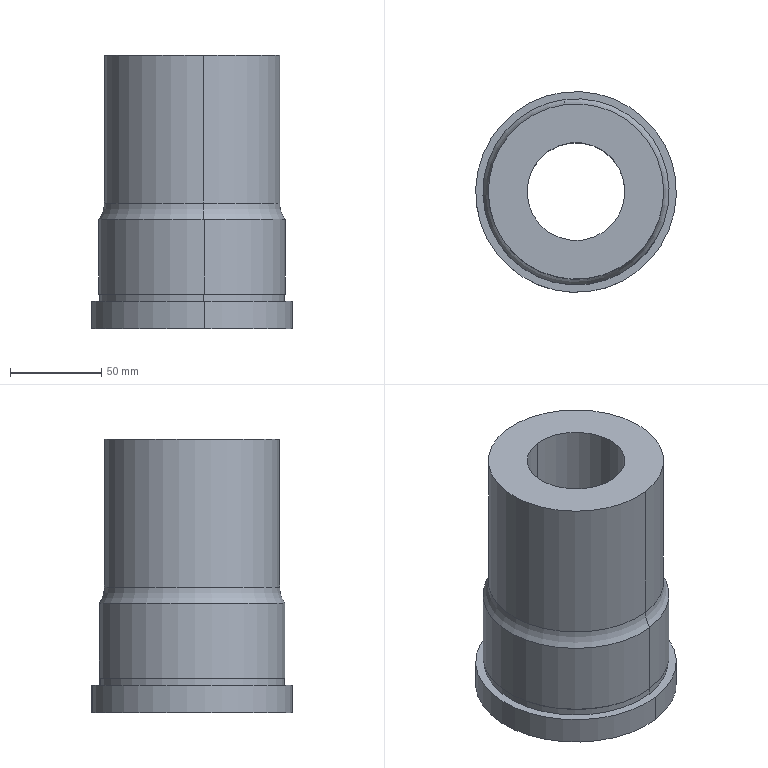Component | SolidWorks | 2-1 | 1 solid | 19 faces | box 110 x 110 x 150 mm | volume 797623 mm3 | cylinder 12 | plane 5 | torus 2 | commonest cylinder face diameters 101 x2 60.5 x2 96.05 x2 102 x2 110 x2 53.65 x2
STEP:
#1=COLOUR_RGB('',0.7922,0.8196,0.9333);
#2=FILL_AREA_STYLE_COLOUR('',#1);
#3=FILL_AREA_STYLE('',(#2));
#4=SURFACE_STYLE_FILL_AREA(#3);
#5=SURFACE_SIDE_STYLE('',(#4));
#6=SURFACE_STYLE_USAGE(.BOTH.,#5);
#7=PRESENTATION_STYLE_ASSIGNMENT((#6));
#8=CARTESIAN_POINT('',(-0.2594,1.991,-7.323));
#9=VERTEX_POINT('',#8);
#10=CARTESIAN_POINT('',(-0.2443,1.875,-6.97));
#11=VERTEX_POINT('',#10);
#12=CARTESIAN_POINT('',(-0.3206,2.461,-6.97));
#13=DIRECTION('',(-0.9916,-0.1292,0.));
#14=DIRECTION('',(-0.1292,0.9916,0.));
#15=AXIS2_PLACEMENT_3D('',#12,#13,#14);
#16=CIRCLE('',#15,0.5906);
#17=EDGE_CURVE('',#9,#11,#16,.T.);
#18=ORIENTED_EDGE('',*,*,#17,.F.);
#19=CARTESIAN_POINT('',(0.2594,-1.991,-7.323));
#20=VERTEX_POINT('',#19);
#21=CARTESIAN_POINT('',(-0.,0.,-7.323));
#22=DIRECTION('',(0.,0.,1.));
#23=DIRECTION('',(-0.1292,0.9916,0.));
#24=AXIS2_PLACEMENT_3D('',#21,#22,#23);
#25=CIRCLE('',#24,2.008);
#26=EDGE_CURVE('',#9,#20,#25,.T.);
#27=ORIENTED_EDGE('',*,*,#26,.T.);
#28=CARTESIAN_POINT('',(0.2443,-1.875,-6.97));
#29=VERTEX_POINT('',#28);
#30=CARTESIAN_POINT('',(0.3206,-2.461,-6.97));
#31=DIRECTION('',(0.9916,0.1292,-0.));
#32=DIRECTION('',(0.1292,-0.9916,0.));
#33=AXIS2_PLACEMENT_3D('',#30,#31,#32);
#34=CIRCLE('',#33,0.5906);
#35=EDGE_CURVE('',#20,#29,#34,.T.);
#36=ORIENTED_EDGE('',*,*,#35,.T.);
#37=CARTESIAN_POINT('',(-0.,0.,-6.97));
#38=DIRECTION('',(0.,0.,1.));
#39=DIRECTION('',(0.1292,-0.9916,0.));
#40=AXIS2_PLACEMENT_3D('',#37,#38,#39);
#41=CIRCLE('',#40,1.891);
#42=EDGE_CURVE('',#11,#29,#41,.T.);
#43=ORIENTED_EDGE('',*,*,#42,.F.);
#44=EDGE_LOOP('',(#18,#27,#36,#43));
#45=FACE_OUTER_BOUND('',#44,.T.);
#46=CARTESIAN_POINT('',(-0.,0.,-6.97));
#47=DIRECTION('',(-0.,-0.,-1.));
#48=DIRECTION('',(0.1292,-0.9916,0.));
#49=AXIS2_PLACEMENT_3D('',#46,#47,#48);
#50=TOROIDAL_SURFACE('',#49,2.481,0.5906);
#51=ADVANCED_FACE('',(#45),#50,.F.);
#52=CARTESIAN_POINT('',(-0.2569,1.972,-8.937));
#53=VERTEX_POINT('',#52);
#54=CARTESIAN_POINT('',(-0.2569,1.972,-9.094));
#55=VERTEX_POINT('',#54);
#56=CARTESIAN_POINT('',(-0.2569,1.972,-8.937));
#57=DIRECTION('',(-0.,-0.,-1.));
#58=VECTOR('',#57,39.37);
#59=LINE('',#56,#58);
#60=EDGE_CURVE('',#53,#55,#59,.T.);
#61=ORIENTED_EDGE('',*,*,#60,.F.);
#62=CARTESIAN_POINT('',(0.2569,-1.972,-8.937));
#63=VERTEX_POINT('',#62);
#64=CARTESIAN_POINT('',(-0.,-0.,-8.937));
#65=DIRECTION('',(0.,0.,1.));
#66=DIRECTION('',(-0.1292,0.9916,0.));
#67=AXIS2_PLACEMENT_3D('',#64,#65,#66);
#68=CIRCLE('',#67,1.988);
#69=EDGE_CURVE('',#63,#53,#68,.T.);
#70=ORIENTED_EDGE('',*,*,#69,.F.);
#71=CARTESIAN_POINT('',(0.2569,-1.972,-9.094));
#72=VERTEX_POINT('',#71);
#73=CARTESIAN_POINT('',(0.2569,-1.972,-8.937));
#74=DIRECTION('',(-0.,-0.,-1.));
#75=VECTOR('',#74,39.37);
#76=LINE('',#73,#75);
#77=EDGE_CURVE('',#63,#72,#76,.T.);
#78=ORIENTED_EDGE('',*,*,#77,.T.);
#79=CARTESIAN_POINT('',(-0.,-0.,-9.094));
#80=DIRECTION('',(0.,0.,1.));
#81=DIRECTION('',(-0.1292,0.9916,0.));
#82=AXIS2_PLACEMENT_3D('',#79,#80,#81);
#83=CIRCLE('',#82,1.988);
#84=EDGE_CURVE('',#72,#55,#83,.T.);
#85=ORIENTED_EDGE('',*,*,#84,.T.);
#86=EDGE_LOOP('',(#61,#70,#78,#85));
#87=FACE_OUTER_BOUND('',#86,.T.);
#88=CARTESIAN_POINT('',(-0.,-0.,-8.937));
#89=DIRECTION('',(-0.,-0.,-1.));
#90=DIRECTION('',(0.1292,-0.9916,0.));
#91=AXIS2_PLACEMENT_3D('',#88,#89,#90);
#92=CYLINDRICAL_SURFACE('',#91,1.988);
#93=ADVANCED_FACE('',(#87),#92,.T.);
#94=ORIENTED_EDGE('',*,*,#69,.T.);
#95=CARTESIAN_POINT('',(-0.,-0.,-8.937));
#96=DIRECTION('',(0.,0.,1.));
#97=DIRECTION('',(-0.1292,0.9916,0.));
#98=AXIS2_PLACEMENT_3D('',#95,#96,#97);
#99=CIRCLE('',#98,1.988);
#100=EDGE_CURVE('',#53,#63,#99,.T.);
#101=ORIENTED_EDGE('',*,*,#100,.T.);
#102=EDGE_LOOP('',(#94,#101));
#103=FACE_BOUND('',#102,.T.);
#104=CARTESIAN_POINT('',(-0.2594,1.991,-8.937));
#105=VERTEX_POINT('',#104);
#106=CARTESIAN_POINT('',(0.2594,-1.991,-8.937));
#107=VERTEX_POINT('',#106);
#108=CARTESIAN_POINT('',(-0.,-0.,-8.937));
#109=DIRECTION('',(0.,0.,1.));
#110=DIRECTION('',(-0.1292,0.9916,0.));
#111=AXIS2_PLACEMENT_3D('',#108,#109,#110);
#112=CIRCLE('',#111,2.008);
#113=EDGE_CURVE('',#105,#107,#112,.T.);
#114=ORIENTED_EDGE('',*,*,#113,.F.);
#115=CARTESIAN_POINT('',(-0.,-0.,-8.937));
#116=DIRECTION('',(0.,0.,1.));
#117=DIRECTION('',(-0.1292,0.9916,0.));
#118=AXIS2_PLACEMENT_3D('',#115,#116,#117);
#119=CIRCLE('',#118,2.008);
#120=EDGE_CURVE('',#107,#105,#119,.T.);
#121=ORIENTED_EDGE('',*,*,#120,.F.);
#122=EDGE_LOOP('',(#114,#121));
#123=FACE_OUTER_BOUND('',#122,.T.);
#124=CARTESIAN_POINT('',(-0.,-0.,-8.937));
#125=DIRECTION('',(0.,0.,1.));
#126=DIRECTION('',(-0.1292,0.9916,-0.));
#127=AXIS2_PLACEMENT_3D('',#124,#125,#126);
#128=PLANE('',#127);
#129=ADVANCED_FACE('',(#103,#123),#128,.F.);
#130=CARTESIAN_POINT('',(-0.1539,1.181,-7.913));
#131=VERTEX_POINT('',#130);
#132=CARTESIAN_POINT('',(-0.1539,1.181,-9.685));
#133=VERTEX_POINT('',#132);
#134=CARTESIAN_POINT('',(-0.1539,1.181,-7.913));
#135=DIRECTION('',(-0.,-0.,-1.));
#136=VECTOR('',#135,39.37);
#137=LINE('',#134,#136);
#138=EDGE_CURVE('',#131,#133,#137,.T.);
#139=ORIENTED_EDGE('',*,*,#138,.F.);
#140=CARTESIAN_POINT('',(0.1539,-1.181,-7.913));
#141=VERTEX_POINT('',#140);
#142=CARTESIAN_POINT('',(-0.,-0.,-7.913));
#143=DIRECTION('',(-0.,-0.,-1.));
#144=DIRECTION('',(0.1292,-0.9916,0.));
#145=AXIS2_PLACEMENT_3D('',#142,#143,#144);
#146=CIRCLE('',#145,1.191);
#147=EDGE_CURVE('',#141,#131,#146,.T.);
#148=ORIENTED_EDGE('',*,*,#147,.F.);
#149=CARTESIAN_POINT('',(0.1539,-1.181,-9.685));
#150=VERTEX_POINT('',#149);
#151=CARTESIAN_POINT('',(0.1539,-1.181,-7.913));
#152=DIRECTION('',(-0.,-0.,-1.));
#153=VECTOR('',#152,39.37);
#154=LINE('',#151,#153);
#155=EDGE_CURVE('',#141,#150,#154,.T.);
#156=ORIENTED_EDGE('',*,*,#155,.T.);
#157=CARTESIAN_POINT('',(-0.,-0.,-9.685));
#158=DIRECTION('',(-0.,-0.,-1.));
#159=DIRECTION('',(0.1292,-0.9916,0.));
#160=AXIS2_PLACEMENT_3D('',#157,#158,#159);
#161=CIRCLE('',#160,1.191);
#162=EDGE_CURVE('',#150,#133,#161,.T.);
#163=ORIENTED_EDGE('',*,*,#162,.T.);
#164=EDGE_LOOP('',(#139,#148,#156,#163));
#165=FACE_OUTER_BOUND('',#164,.T.);
#166=CARTESIAN_POINT('',(-0.,-0.,-7.913));
#167=DIRECTION('',(-0.,-0.,-1.));
#168=DIRECTION('',(0.1292,-0.9916,0.));
#169=AXIS2_PLACEMENT_3D('',#166,#167,#168);
#170=CYLINDRICAL_SURFACE('',#169,1.191);
#171=ADVANCED_FACE('',(#165),#170,.F.);
#172=CARTESIAN_POINT('',(-0.1364,1.047,-7.913));
#173=VERTEX_POINT('',#172);
#174=CARTESIAN_POINT('',(0.1364,-1.047,-7.913));
#175=VERTEX_POINT('',#174);
#176=CARTESIAN_POINT('',(-0.,-0.,-7.913));
#177=DIRECTION('',(0.,0.,1.));
#178=DIRECTION('',(0.1292,-0.9916,0.));
#179=AXIS2_PLACEMENT_3D('',#176,#177,#178);
#180=CIRCLE('',#179,1.056);
#181=EDGE_CURVE('',#173,#175,#180,.T.);
#182=ORIENTED_EDGE('',*,*,#181,.T.);
#183=CARTESIAN_POINT('',(-0.,-0.,-7.913));
#184=DIRECTION('',(0.,0.,1.));
#185=DIRECTION('',(0.1292,-0.9916,0.));
#186=AXIS2_PLACEMENT_3D('',#183,#184,#185);
#187=CIRCLE('',#186,1.056);
#188=EDGE_CURVE('',#175,#173,#187,.T.);
#189=ORIENTED_EDGE('',*,*,#188,.T.);
#190=EDGE_LOOP('',(#182,#189));
#191=FACE_BOUND('',#190,.T.);
#192=ORIENTED_EDGE('',*,*,#147,.T.);
#193=CARTESIAN_POINT('',(-0.,-0.,-7.913));
#194=DIRECTION('',(-0.,-0.,-1.));
#195=DIRECTION('',(0.1292,-0.9916,0.));
#196=AXIS2_PLACEMENT_3D('',#193,#194,#195);
#197=CIRCLE('',#196,1.191);
#198=EDGE_CURVE('',#131,#141,#197,.T.);
#199=ORIENTED_EDGE('',*,*,#198,.T.);
#200=EDGE_LOOP('',(#192,#199));
#201=FACE_OUTER_BOUND('',#200,.T.);
#202=CARTESIAN_POINT('',(-0.,-0.,-7.913));
#203=DIRECTION('',(-0.,-0.,-1.));
#204=DIRECTION('',(-0.9916,-0.1292,0.));
#205=AXIS2_PLACEMENT_3D('',#202,#203,#204);
#206=PLANE('',#205);
#207=ADVANCED_FACE('',(#191,#201),#206,.T.);
#208=CARTESIAN_POINT('',(0.2443,-1.875,-3.78));
#209=VERTEX_POINT('',#208);
#210=CARTESIAN_POINT('',(0.2443,-1.875,-3.78));
#211=DIRECTION('',(0.,0.,1.));
#212=VECTOR('',#211,39.37);
#213=LINE('',#210,#212);
#214=EDGE_CURVE('',#29,#209,#213,.T.);
#215=ORIENTED_EDGE('',*,*,#214,.F.);
#216=CARTESIAN_POINT('',(-0.,0.,-6.97));
#217=DIRECTION('',(0.,0.,1.));
#218=DIRECTION('',(0.1292,-0.9916,0.));
#219=AXIS2_PLACEMENT_3D('',#216,#217,#218);
#220=CIRCLE('',#219,1.891);
#221=EDGE_CURVE('',#29,#11,#220,.T.);
#222=ORIENTED_EDGE('',*,*,#221,.T.);
#223=CARTESIAN_POINT('',(-0.2443,1.875,-3.78));
#224=VERTEX_POINT('',#223);
#225=CARTESIAN_POINT('',(-0.2443,1.875,-3.78));
#226=DIRECTION('',(0.,0.,1.));
#227=VECTOR('',#226,39.37);
#228=LINE('',#225,#227);
#229=EDGE_CURVE('',#11,#224,#228,.T.);
#230=ORIENTED_EDGE('',*,*,#229,.T.);
#231=CARTESIAN_POINT('',(-0.,0.,-3.78));
#232=DIRECTION('',(0.,0.,1.));
#233=DIRECTION('',(-0.1292,0.9916,0.));
#234=AXIS2_PLACEMENT_3D('',#231,#232,#233);
#235=CIRCLE('',#234,1.891);
#236=EDGE_CURVE('',#209,#224,#235,.T.);
#237=ORIENTED_EDGE('',*,*,#236,.F.);
#238=EDGE_LOOP('',(#215,#222,#230,#237));
#239=FACE_OUTER_BOUND('',#238,.T.);
#240=CARTESIAN_POINT('',(-0.,0.,-3.78));
#241=DIRECTION('',(0.,0.,1.));
#242=DIRECTION('',(-0.1292,0.9916,0.));
#243=AXIS2_PLACEMENT_3D('',#240,#241,#242);
#244=CYLINDRICAL_SURFACE('',#243,1.891);
#245=ADVANCED_FACE('',(#239),#244,.T.);
#246=CARTESIAN_POINT('',(0.2594,-1.991,-3.78));
#247=DIRECTION('',(0.,0.,1.));
#248=VECTOR('',#247,39.37);
#249=LINE('',#246,#248);
#250=EDGE_CURVE('',#107,#20,#249,.T.);
#251=ORIENTED_EDGE('',*,*,#250,.F.);
#252=ORIENTED_EDGE('',*,*,#120,.T.);
#253=CARTESIAN_POINT('',(-0.2594,1.991,-3.78));
#254=DIRECTION('',(0.,0.,1.));
#255=VECTOR('',#254,39.37);
#256=LINE('',#253,#255);
#257=EDGE_CURVE('',#105,#9,#256,.T.);
#258=ORIENTED_EDGE('',*,*,#257,.T.);
#259=CARTESIAN_POINT('',(-0.,0.,-7.323));
#260=DIRECTION('',(0.,0.,1.));
#261=DIRECTION('',(-0.1292,0.9916,0.));
#262=AXIS2_PLACEMENT_3D('',#259,#260,#261);
#263=CIRCLE('',#262,2.008);
#264=EDGE_CURVE('',#20,#9,#263,.T.);
#265=ORIENTED_EDGE('',*,*,#264,.F.);
#266=EDGE_LOOP('',(#251,#252,#258,#265));
#267=FACE_OUTER_BOUND('',#266,.T.);
#268=CARTESIAN_POINT('',(-0.,0.,-3.78));
#269=DIRECTION('',(0.,0.,1.));
#270=DIRECTION('',(-0.1292,0.9916,0.));
#271=AXIS2_PLACEMENT_3D('',#268,#269,#270);
#272=CYLINDRICAL_SURFACE('',#271,2.008);
#273=ADVANCED_FACE('',(#267),#272,.T.);
#274=ORIENTED_EDGE('',*,*,#84,.F.);
#275=CARTESIAN_POINT('',(-0.,-0.,-9.094));
#276=DIRECTION('',(0.,0.,1.));
#277=DIRECTION('',(-0.1292,0.9916,0.));
#278=AXIS2_PLACEMENT_3D('',#275,#276,#277);
#279=CIRCLE('',#278,1.988);
#280=EDGE_CURVE('',#55,#72,#279,.T.);
#281=ORIENTED_EDGE('',*,*,#280,.F.);
#282=EDGE_LOOP('',(#274,#281));
#283=FACE_BOUND('',#282,.T.);
#284=CARTESIAN_POINT('',(-0.2797,2.147,-9.094));
#285=VERTEX_POINT('',#284);
#286=CARTESIAN_POINT('',(0.2797,-2.147,-9.094));
#287=VERTEX_POINT('',#286);
#288=CARTESIAN_POINT('',(-0.,-0.,-9.094));
#289=DIRECTION('',(0.,0.,1.));
#290=DIRECTION('',(-0.1292,0.9916,0.));
#291=AXIS2_PLACEMENT_3D('',#288,#289,#290);
#292=CIRCLE('',#291,2.165);
#293=EDGE_CURVE('',#285,#287,#292,.T.);
#294=ORIENTED_EDGE('',*,*,#293,.T.);
#295=CARTESIAN_POINT('',(-0.,-0.,-9.094));
#296=DIRECTION('',(0.,0.,1.));
#297=DIRECTION('',(-0.1292,0.9916,0.));
#298=AXIS2_PLACEMENT_3D('',#295,#296,#297);
#299=CIRCLE('',#298,2.165);
#300=EDGE_CURVE('',#287,#285,#299,.T.);
#301=ORIENTED_EDGE('',*,*,#300,.T.);
#302=EDGE_LOOP('',(#294,#301));
#303=FACE_OUTER_BOUND('',#302,.T.);
#304=CARTESIAN_POINT('',(-2.147,-0.2797,-9.094));
#305=DIRECTION('',(0.,0.,1.));
#306=DIRECTION('',(-0.1292,0.9916,-0.));
#307=AXIS2_PLACEMENT_3D('',#304,#305,#306);
#308=PLANE('',#307);
#309=ADVANCED_FACE('',(#283,#303),#308,.T.);
#310=CARTESIAN_POINT('',(0.2797,-2.147,-9.685));
#311=VERTEX_POINT('',#310);
#312=CARTESIAN_POINT('',(0.2797,-2.147,-3.78));
#313=DIRECTION('',(0.,0.,1.));
#314=VECTOR('',#313,39.37);
#315=LINE('',#312,#314);
#316=EDGE_CURVE('',#311,#287,#315,.T.);
#317=ORIENTED_EDGE('',*,*,#316,.F.);
#318=CARTESIAN_POINT('',(-0.2797,2.147,-9.685));
#319=VERTEX_POINT('',#318);
#320=CARTESIAN_POINT('',(-0.,-0.,-9.685));
#321=DIRECTION('',(0.,0.,1.));
#322=DIRECTION('',(-0.1292,0.9916,0.));
#323=AXIS2_PLACEMENT_3D('',#320,#321,#322);
#324=CIRCLE('',#323,2.165);
#325=EDGE_CURVE('',#311,#319,#324,.T.);
#326=ORIENTED_EDGE('',*,*,#325,.T.);
#327=CARTESIAN_POINT('',(-0.2797,2.147,-3.78));
#328=DIRECTION('',(0.,0.,1.));
#329=VECTOR('',#328,39.37);
#330=LINE('',#327,#329);
#331=EDGE_CURVE('',#319,#285,#330,.T.);
#332=ORIENTED_EDGE('',*,*,#331,.T.);
#333=ORIENTED_EDGE('',*,*,#300,.F.);
#334=EDGE_LOOP('',(#317,#326,#332,#333));
#335=FACE_OUTER_BOUND('',#334,.T.);
#336=CARTESIAN_POINT('',(-0.,0.,-3.78));
#337=DIRECTION('',(0.,0.,1.));
#338=DIRECTION('',(-0.1292,0.9916,0.));
#339=AXIS2_PLACEMENT_3D('',#336,#337,#338);
#340=CYLINDRICAL_SURFACE('',#339,2.165);
#341=ADVANCED_FACE('',(#335),#340,.T.);
#342=ORIENTED_EDGE('',*,*,#162,.F.);
#343=CARTESIAN_POINT('',(-0.,-0.,-9.685));
#344=DIRECTION('',(-0.,-0.,-1.));
#345=DIRECTION('',(0.1292,-0.9916,0.));
#346=AXIS2_PLACEMENT_3D('',#343,#344,#345);
#347=CIRCLE('',#346,1.191);
#348=EDGE_CURVE('',#133,#150,#347,.T.);
#349=ORIENTED_EDGE('',*,*,#348,.F.);
#350=EDGE_LOOP('',(#342,#349));
#351=FACE_BOUND('',#350,.T.);
#352=CARTESIAN_POINT('',(-0.,-0.,-9.685));
#353=DIRECTION('',(0.,0.,1.));
#354=DIRECTION('',(-0.1292,0.9916,0.));
#355=AXIS2_PLACEMENT_3D('',#352,#353,#354);
#356=CIRCLE('',#355,2.165);
#357=EDGE_CURVE('',#319,#311,#356,.T.);
#358=ORIENTED_EDGE('',*,*,#357,.F.);
#359=ORIENTED_EDGE('',*,*,#325,.F.);
#360=EDGE_LOOP('',(#358,#359));
#361=FACE_OUTER_BOUND('',#360,.T.);
#362=CARTESIAN_POINT('',(-0.,-0.,-9.685));
#363=DIRECTION('',(-0.,-0.,-1.));
#364=DIRECTION('',(-0.9916,-0.1292,0.));
#365=AXIS2_PLACEMENT_3D('',#362,#363,#364);
#366=PLANE('',#365);
#367=ADVANCED_FACE('',(#351,#361),#366,.T.);
#368=CARTESIAN_POINT('',(-0.1364,1.047,-3.78));
#369=VERTEX_POINT('',#368);
#370=CARTESIAN_POINT('',(0.1364,-1.047,-3.78));
#371=VERTEX_POINT('',#370);
#372=CARTESIAN_POINT('',(-0.,0.,-3.78));
#373=DIRECTION('',(0.,0.,1.));
#374=DIRECTION('',(-0.1292,0.9916,0.));
#375=AXIS2_PLACEMENT_3D('',#372,#373,#374);
#376=CIRCLE('',#375,1.056);
#377=EDGE_CURVE('',#369,#371,#376,.T.);
#378=ORIENTED_EDGE('',*,*,#377,.F.);
#379=CARTESIAN_POINT('',(-0.,0.,-3.78));
#380=DIRECTION('',(0.,0.,1.));
#381=DIRECTION('',(-0.1292,0.9916,0.));
#382=AXIS2_PLACEMENT_3D('',#379,#380,#381);
#383=CIRCLE('',#382,1.056);
#384=EDGE_CURVE('',#371,#369,#383,.T.);
#385=ORIENTED_EDGE('',*,*,#384,.F.);
#386=EDGE_LOOP('',(#378,#385));
#387=FACE_BOUND('',#386,.T.);
#388=CARTESIAN_POINT('',(-0.,0.,-3.78));
#389=DIRECTION('',(0.,0.,1.));
#390=DIRECTION('',(-0.1292,0.9916,0.));
#391=AXIS2_PLACEMENT_3D('',#388,#389,#390);
#392=CIRCLE('',#391,1.891);
#393=EDGE_CURVE('',#224,#209,#392,.T.);
#394=ORIENTED_EDGE('',*,*,#393,.T.);
#395=ORIENTED_EDGE('',*,*,#236,.T.);
#396=EDGE_LOOP('',(#394,#395));
#397=FACE_OUTER_BOUND('',#396,.T.);
#398=CARTESIAN_POINT('',(-1.875,-0.2443,-3.78));
#399=DIRECTION('',(0.,0.,1.));
#400=DIRECTION('',(-0.1292,0.9916,-0.));
#401=AXIS2_PLACEMENT_3D('',#398,#399,#400);
#402=PLANE('',#401);
#403=ADVANCED_FACE('',(#387,#397),#402,.T.);
#404=CARTESIAN_POINT('',(0.1364,-1.047,-9.685));
#405=DIRECTION('',(0.,0.,1.));
#406=VECTOR('',#405,39.37);
#407=LINE('',#404,#406);
#408=EDGE_CURVE('',#175,#371,#407,.T.);
#409=ORIENTED_EDGE('',*,*,#408,.F.);
#410=ORIENTED_EDGE('',*,*,#181,.F.);
#411=CARTESIAN_POINT('',(-0.1364,1.047,-9.685));
#412=DIRECTION('',(0.,0.,1.));
#413=VECTOR('',#412,39.37);
#414=LINE('',#411,#413);
#415=EDGE_CURVE('',#173,#369,#414,.T.);
#416=ORIENTED_EDGE('',*,*,#415,.T.);
#417=ORIENTED_EDGE('',*,*,#377,.T.);
#418=EDGE_LOOP('',(#409,#410,#416,#417));
#419=FACE_OUTER_BOUND('',#418,.T.);
#420=CARTESIAN_POINT('',(-0.,-0.,-9.685));
#421=DIRECTION('',(0.,0.,1.));
#422=DIRECTION('',(-0.1292,0.9916,0.));
#423=AXIS2_PLACEMENT_3D('',#420,#421,#422);
#424=CYLINDRICAL_SURFACE('',#423,1.056);
#425=ADVANCED_FACE('',(#419),#424,.F.);
#426=ORIENTED_EDGE('',*,*,#188,.F.);
#427=ORIENTED_EDGE('',*,*,#408,.T.);
#428=ORIENTED_EDGE('',*,*,#384,.T.);
#429=ORIENTED_EDGE('',*,*,#415,.F.);
#430=EDGE_LOOP('',(#426,#427,#428,#429));
#431=FACE_OUTER_BOUND('',#430,.T.);
#432=CARTESIAN_POINT('',(-0.,-0.,-9.685));
#433=DIRECTION('',(0.,0.,1.));
#434=DIRECTION('',(-0.1292,0.9916,0.));
#435=AXIS2_PLACEMENT_3D('',#432,#433,#434);
#436=CYLINDRICAL_SURFACE('',#435,1.056);
#437=ADVANCED_FACE('',(#431),#436,.F.);
#438=ORIENTED_EDGE('',*,*,#357,.T.);
#439=ORIENTED_EDGE('',*,*,#316,.T.);
#440=ORIENTED_EDGE('',*,*,#293,.F.);
#441=ORIENTED_EDGE('',*,*,#331,.F.);
#442=EDGE_LOOP('',(#438,#439,#440,#441));
#443=FACE_OUTER_BOUND('',#442,.T.);
#444=CARTESIAN_POINT('',(-0.,0.,-3.78));
#445=DIRECTION('',(0.,0.,1.));
#446=DIRECTION('',(-0.1292,0.9916,0.));
#447=AXIS2_PLACEMENT_3D('',#444,#445,#446);
#448=CYLINDRICAL_SURFACE('',#447,2.165);
#449=ADVANCED_FACE('',(#443),#448,.T.);
#450=ORIENTED_EDGE('',*,*,#113,.T.);
#451=ORIENTED_EDGE('',*,*,#250,.T.);
#452=ORIENTED_EDGE('',*,*,#26,.F.);
#453=ORIENTED_EDGE('',*,*,#257,.F.);
#454=EDGE_LOOP('',(#450,#451,#452,#453));
#455=FACE_OUTER_BOUND('',#454,.T.);
#456=CARTESIAN_POINT('',(-0.,0.,-3.78));
#457=DIRECTION('',(0.,0.,1.));
#458=DIRECTION('',(-0.1292,0.9916,0.));
#459=AXIS2_PLACEMENT_3D('',#456,#457,#458);
#460=CYLINDRICAL_SURFACE('',#459,2.008);
#461=ADVANCED_FACE('',(#455),#460,.T.);
#462=ORIENTED_EDGE('',*,*,#42,.T.);
#463=ORIENTED_EDGE('',*,*,#214,.T.);
#464=ORIENTED_EDGE('',*,*,#393,.F.);
#465=ORIENTED_EDGE('',*,*,#229,.F.);
#466=EDGE_LOOP('',(#462,#463,#464,#465));
#467=FACE_OUTER_BOUND('',#466,.T.);
#468=CARTESIAN_POINT('',(-0.,0.,-3.78));
#469=DIRECTION('',(0.,0.,1.));
#470=DIRECTION('',(-0.1292,0.9916,0.));
#471=AXIS2_PLACEMENT_3D('',#468,#469,#470);
#472=CYLINDRICAL_SURFACE('',#471,1.891);
#473=ADVANCED_FACE('',(#467),#472,.T.);
#474=ORIENTED_EDGE('',*,*,#198,.F.);
#475=ORIENTED_EDGE('',*,*,#138,.T.);
#476=ORIENTED_EDGE('',*,*,#348,.T.);
#477=ORIENTED_EDGE('',*,*,#155,.F.);
#478=EDGE_LOOP('',(#474,#475,#476,#477));
#479=FACE_OUTER_BOUND('',#478,.T.);
#480=CARTESIAN_POINT('',(-0.,-0.,-7.913));
#481=DIRECTION('',(-0.,-0.,-1.));
#482=DIRECTION('',(0.1292,-0.9916,0.));
#483=AXIS2_PLACEMENT_3D('',#480,#481,#482);
#484=CYLINDRICAL_SURFACE('',#483,1.191);
#485=ADVANCED_FACE('',(#479),#484,.F.);
#486=ORIENTED_EDGE('',*,*,#100,.F.);
#487=ORIENTED_EDGE('',*,*,#60,.T.);
#488=ORIENTED_EDGE('',*,*,#280,.T.);
#489=ORIENTED_EDGE('',*,*,#77,.F.);
#490=EDGE_LOOP('',(#486,#487,#488,#489));
#491=FACE_OUTER_BOUND('',#490,.T.);
#492=CARTESIAN_POINT('',(-0.,-0.,-8.937));
#493=DIRECTION('',(-0.,-0.,-1.));
#494=DIRECTION('',(0.1292,-0.9916,0.));
#495=AXIS2_PLACEMENT_3D('',#492,#493,#494);
#496=CYLINDRICAL_SURFACE('',#495,1.988);
#497=ADVANCED_FACE('',(#491),#496,.T.);
#498=ORIENTED_EDGE('',*,*,#264,.T.);
#499=ORIENTED_EDGE('',*,*,#17,.T.);
#500=ORIENTED_EDGE('',*,*,#221,.F.);
#501=ORIENTED_EDGE('',*,*,#35,.F.);
#502=EDGE_LOOP('',(#498,#499,#500,#501));
#503=FACE_OUTER_BOUND('',#502,.T.);
#504=CARTESIAN_POINT('',(-0.,0.,-6.97));
#505=DIRECTION('',(-0.,-0.,-1.));
#506=DIRECTION('',(0.1292,-0.9916,0.));
#507=AXIS2_PLACEMENT_3D('',#504,#505,#506);
#508=TOROIDAL_SURFACE('',#507,2.481,0.5906);
#509=ADVANCED_FACE('',(#503),#508,.F.);
#510=CLOSED_SHELL('',(#51,#93,#129,#171,#207,#245,#273,#309,#341,#367,#403,#425,#437,#449,#461,#473,#485,#497,#509));
#511=MANIFOLD_SOLID_BREP('',#510);
#512=STYLED_ITEM('',(#7),#511);
#513=PRESENTATION_LAYER_ASSIGNMENT('','',(#512));
#514=(LENGTH_UNIT()NAMED_UNIT(*)SI_UNIT($,.METRE.));
#515=LENGTH_MEASURE_WITH_UNIT(LENGTH_MEASURE(0.0254),#514);
#516=DIMENSIONAL_EXPONENTS(1.,0.,0.,0.,0.,0.,0.);
#517=(CONVERSION_BASED_UNIT('',#515)LENGTH_UNIT()NAMED_UNIT(#516));
#518=UNCERTAINTY_MEASURE_WITH_UNIT(LENGTH_MEASURE(0.00001),#517,'','');
#519=(NAMED_UNIT(*)PLANE_ANGLE_UNIT()SI_UNIT($,.RADIAN.));
#520=(NAMED_UNIT(*)SI_UNIT($,.STERADIAN.)SOLID_ANGLE_UNIT());
#521=(GEOMETRIC_REPRESENTATION_CONTEXT(3)GLOBAL_UNCERTAINTY_ASSIGNED_CONTEXT((#518))GLOBAL_UNIT_ASSIGNED_CONTEXT((#517,#519,#520))REPRESENTATION_CONTEXT('',''));
#522=MECHANICAL_DESIGN_GEOMETRIC_PRESENTATION_REPRESENTATION('',(#512),#521);
#523=CARTESIAN_POINT('',(0.,0.,0.));
#524=DIRECTION('',(0.,0.,1.));
#525=DIRECTION('',(1.,0.,0.));
#526=AXIS2_PLACEMENT_3D('',#523,#524,#525);
#527=(LENGTH_UNIT()NAMED_UNIT(*)SI_UNIT($,.METRE.));
#528=LENGTH_MEASURE_WITH_UNIT(LENGTH_MEASURE(0.0254),#527);
#529=DIMENSIONAL_EXPONENTS(1.,0.,0.,0.,0.,0.,0.);
#530=(CONVERSION_BASED_UNIT('',#528)LENGTH_UNIT()NAMED_UNIT(#529));
#531=UNCERTAINTY_MEASURE_WITH_UNIT(LENGTH_MEASURE(0.00001),#530,'','');
#532=(NAMED_UNIT(*)PLANE_ANGLE_UNIT()SI_UNIT($,.RADIAN.));
#533=(NAMED_UNIT(*)SI_UNIT($,.STERADIAN.)SOLID_ANGLE_UNIT());
#534=(GEOMETRIC_REPRESENTATION_CONTEXT(3)GLOBAL_UNCERTAINTY_ASSIGNED_CONTEXT((#531))GLOBAL_UNIT_ASSIGNED_CONTEXT((#530,#532,#533))REPRESENTATION_CONTEXT('',''));
#535=ADVANCED_BREP_SHAPE_REPRESENTATION('',(#511,#526),#534);